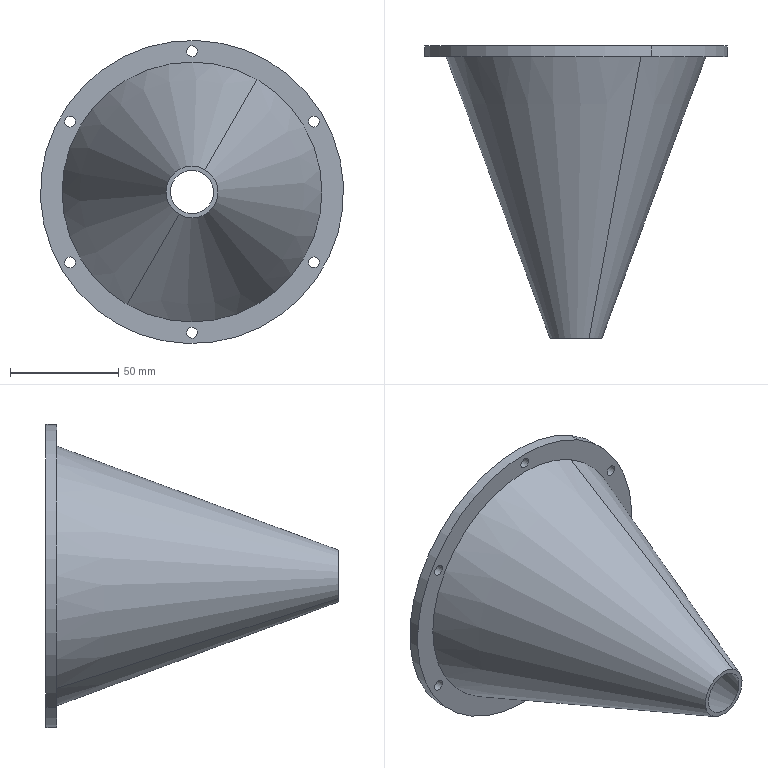Component | SolidWorks | WorkingHeadLowerCover-1 | 1 solid | 21 faces | box 140 x 135 x 140 mm | volume 112383 mm3 | cylinder 14 | cone 4 | plane 3 | commonest cylinder face diameters 5 x12 140 x2
build123d program:
from build123d import *

# Parameters (mm, degrees)
CUT_EXTRUDE1_REACH = 169.407
SKETCH2_R          = 2.5


with BuildPart() as part:
    # Sketch1 → Revolve1 (revolve)
    with BuildSketch(Plane.XY, mode=Mode.PRIVATE) as revolve1_sk:
        Polygon((-109.742, 0), (25.258, 0), (25.258, 12), (-104.742, 60), (-104.742, 70), (-109.742, 70), align=None)
    revolve(revolve1_sk.sketch.rotate(Axis((-109.742, 0, 0), (1, 0, 0)), 90), axis=Axis((-109.742, 0, 0), (1, 0, 0)))

    # Sketch2 → Cut-Extrude1 (cut, up to next)
    with BuildSketch(Plane.ZY.offset(109.742), mode=Mode.PRIVATE) as cut_extrude1_sk1:
        with Locations((0, 65)):
            Circle(SKETCH2_R)
    cut_extrude1_tool1 = extrude(cut_extrude1_sk1.sketch, amount=-CUT_EXTRUDE1_REACH, mode=Mode.PRIVATE) & part.part
    # Sketch2 → Cut-Extrude1 (cut, up to next)
    with BuildSketch(Plane.ZY.offset(109.742), mode=Mode.PRIVATE) as cut_extrude1_sk2:
        with Locations((56.292, 32.5)):
            Circle(SKETCH2_R)
    cut_extrude1_tool2 = extrude(cut_extrude1_sk2.sketch, amount=-CUT_EXTRUDE1_REACH, mode=Mode.PRIVATE) & part.part
    # Sketch2 → Cut-Extrude1 (cut, up to next)
    with BuildSketch(Plane.ZY.offset(109.742), mode=Mode.PRIVATE) as cut_extrude1_sk3:
        with Locations((56.292, -32.5)):
            Circle(SKETCH2_R)
    cut_extrude1_tool3 = extrude(cut_extrude1_sk3.sketch, amount=-CUT_EXTRUDE1_REACH, mode=Mode.PRIVATE) & part.part
    # Sketch2 → Cut-Extrude1 (cut, up to next)
    with BuildSketch(Plane.ZY.offset(109.742), mode=Mode.PRIVATE) as cut_extrude1_sk4:
        with Locations((0, -65)):
            Circle(SKETCH2_R)
    cut_extrude1_tool4 = extrude(cut_extrude1_sk4.sketch, amount=-CUT_EXTRUDE1_REACH, mode=Mode.PRIVATE) & part.part
    # Sketch2 → Cut-Extrude1 (cut, up to next)
    with BuildSketch(Plane.ZY.offset(109.742), mode=Mode.PRIVATE) as cut_extrude1_sk5:
        with Locations((-56.292, -32.5)):
            Circle(SKETCH2_R)
    cut_extrude1_tool5 = extrude(cut_extrude1_sk5.sketch, amount=-CUT_EXTRUDE1_REACH, mode=Mode.PRIVATE) & part.part
    # Sketch2 → Cut-Extrude1 (cut, up to next)
    with BuildSketch(Plane.ZY.offset(109.742), mode=Mode.PRIVATE) as cut_extrude1_sk6:
        with Locations((-56.292, 32.5)):
            Circle(SKETCH2_R)
    cut_extrude1_tool6 = extrude(cut_extrude1_sk6.sketch, amount=-CUT_EXTRUDE1_REACH, mode=Mode.PRIVATE) & part.part
    add(cut_extrude1_tool1.solids().sort_by_distance((-109.742, 65, 0))[0], mode=Mode.SUBTRACT)
    add(cut_extrude1_tool2.solids().sort_by_distance((-109.742, 32.5, 56.292))[0], mode=Mode.SUBTRACT)
    add(cut_extrude1_tool3.solids().sort_by_distance((-109.742, -32.5, 56.292))[0], mode=Mode.SUBTRACT)
    add(cut_extrude1_tool4.solids().sort_by_distance((-109.742, -65, 0))[0], mode=Mode.SUBTRACT)
    add(cut_extrude1_tool5.solids().sort_by_distance((-109.742, -32.5, -56.292))[0], mode=Mode.SUBTRACT)
    add(cut_extrude1_tool6.solids().sort_by_distance((-109.742, 32.5, -56.292))[0], mode=Mode.SUBTRACT)

    # Sketch3 → Cut-Revolve1 (revolve, cut)
    with BuildSketch(Plane(origin=(0, 0, 0), x_dir=(1, 0, 0), z_dir=(0, 1, 0)), mode=Mode.PRIVATE) as cut_revolve1_sk:
        Polygon((-109.742, 0), (25.258, 0), (25.258, 10), (-109.742, 58), align=None)
    revolve(cut_revolve1_sk.sketch.rotate(Axis((-109.742, 0, 0), (1, 0, 0)), 180), axis=Axis((-109.742, 0, 0), (1, 0, 0)), mode=Mode.SUBTRACT)


solid = part.part

# Placed as in the assembly
solid = solid.moved(Location((-5.981, -119.235, 160), (90, -90, 0)))
STEP:
#1=COLOUR_RGB('',0.7922,0.8196,0.9333);
#2=FILL_AREA_STYLE_COLOUR('',#1);
#3=FILL_AREA_STYLE('',(#2));
#4=SURFACE_STYLE_FILL_AREA(#3);
#5=SURFACE_SIDE_STYLE('',(#4));
#6=SURFACE_STYLE_USAGE(.BOTH.,#5);
#7=PRESENTATION_STYLE_ASSIGNMENT((#6));
#8=CARTESIAN_POINT('',(-0.4323,-5.689,5.958));
#9=VERTEX_POINT('',#8);
#10=CARTESIAN_POINT('',(-0.03862,-5.689,6.64));
#11=VERTEX_POINT('',#10);
#12=CARTESIAN_POINT('',(-0.2355,-5.689,6.299));
#13=DIRECTION('',(0.,1.,0.));
#14=DIRECTION('',(0.5,0.,0.866));
#15=AXIS2_PLACEMENT_3D('',#12,#13,#14);
#16=CIRCLE('',#15,0.3937);
#17=EDGE_CURVE('',#9,#11,#16,.T.);
#18=ORIENTED_EDGE('',*,*,#17,.F.);
#19=CARTESIAN_POINT('',(-1.377,-0.3738,4.322));
#20=VERTEX_POINT('',#19);
#21=CARTESIAN_POINT('',(-0.4323,-5.689,5.958));
#22=DIRECTION('',(-0.1675,0.9422,-0.2901));
#23=VECTOR('',#22,39.37);
#24=LINE('',#21,#23);
#25=EDGE_CURVE('',#9,#20,#24,.T.);
#26=ORIENTED_EDGE('',*,*,#25,.T.);
#27=CARTESIAN_POINT('',(0.9063,-0.3738,8.277));
#28=VERTEX_POINT('',#27);
#29=CARTESIAN_POINT('',(-0.2355,-0.3738,6.299));
#30=DIRECTION('',(0.,1.,0.));
#31=DIRECTION('',(0.5,0.,0.866));
#32=AXIS2_PLACEMENT_3D('',#29,#30,#31);
#33=CIRCLE('',#32,2.283);
#34=EDGE_CURVE('',#20,#28,#33,.T.);
#35=ORIENTED_EDGE('',*,*,#34,.T.);
#36=CARTESIAN_POINT('',(-0.03862,-5.689,6.64));
#37=DIRECTION('',(0.1675,0.9422,0.2901));
#38=VECTOR('',#37,39.37);
#39=LINE('',#36,#38);
#40=EDGE_CURVE('',#11,#28,#39,.T.);
#41=ORIENTED_EDGE('',*,*,#40,.F.);
#42=EDGE_LOOP('',(#18,#26,#35,#41));
#43=FACE_OUTER_BOUND('',#42,.T.);
#44=CARTESIAN_POINT('',(-0.2355,-5.689,6.299));
#45=DIRECTION('',(0.,1.,0.));
#46=DIRECTION('',(0.5,0.,0.866));
#47=AXIS2_PLACEMENT_3D('',#44,#45,#46);
#48=CONICAL_SURFACE('',#47,0.3937,0.3416);
#49=ADVANCED_FACE('',(#43),#48,.F.);
#50=CARTESIAN_POINT('',(2.03,-0.5706,5.105));
#51=VERTEX_POINT('',#50);
#52=CARTESIAN_POINT('',(1.932,-0.5706,4.934));
#53=VERTEX_POINT('',#52);
#54=CARTESIAN_POINT('',(1.981,-0.5706,5.02));
#55=DIRECTION('',(0.,-1.,0.));
#56=DIRECTION('',(0.5,0.,0.866));
#57=AXIS2_PLACEMENT_3D('',#54,#55,#56);
#58=CIRCLE('',#57,0.09843);
#59=EDGE_CURVE('',#51,#53,#58,.T.);
#60=ORIENTED_EDGE('',*,*,#59,.T.);
#61=CARTESIAN_POINT('',(1.932,-0.3738,4.934));
#62=VERTEX_POINT('',#61);
#63=CARTESIAN_POINT('',(1.932,-5.689,4.934));
#64=DIRECTION('',(0.,1.,0.));
#65=VECTOR('',#64,39.37);
#66=LINE('',#63,#65);
#67=EDGE_CURVE('',#53,#62,#66,.T.);
#68=ORIENTED_EDGE('',*,*,#67,.T.);
#69=CARTESIAN_POINT('',(2.03,-0.3738,5.105));
#70=VERTEX_POINT('',#69);
#71=CARTESIAN_POINT('',(1.981,-0.3738,5.02));
#72=DIRECTION('',(0.,1.,0.));
#73=DIRECTION('',(0.5,0.,0.866));
#74=AXIS2_PLACEMENT_3D('',#71,#72,#73);
#75=CIRCLE('',#74,0.09843);
#76=EDGE_CURVE('',#62,#70,#75,.T.);
#77=ORIENTED_EDGE('',*,*,#76,.T.);
#78=CARTESIAN_POINT('',(2.03,-5.689,5.105));
#79=DIRECTION('',(0.,1.,0.));
#80=VECTOR('',#79,39.37);
#81=LINE('',#78,#80);
#82=EDGE_CURVE('',#51,#70,#81,.T.);
#83=ORIENTED_EDGE('',*,*,#82,.F.);
#84=EDGE_LOOP('',(#60,#68,#77,#83));
#85=FACE_OUTER_BOUND('',#84,.T.);
#86=CARTESIAN_POINT('',(1.981,-5.689,5.02));
#87=DIRECTION('',(0.,1.,0.));
#88=DIRECTION('',(0.5,0.,0.866));
#89=AXIS2_PLACEMENT_3D('',#86,#87,#88);
#90=CYLINDRICAL_SURFACE('',#89,0.09843);
#91=ADVANCED_FACE('',(#85),#90,.F.);
#92=CARTESIAN_POINT('',(-0.1863,-0.5706,3.825));
#93=VERTEX_POINT('',#92);
#94=CARTESIAN_POINT('',(-0.2847,-0.5706,3.655));
#95=VERTEX_POINT('',#94);
#96=CARTESIAN_POINT('',(-0.2355,-0.5706,3.74));
#97=DIRECTION('',(0.,-1.,0.));
#98=DIRECTION('',(0.5,0.,0.866));
#99=AXIS2_PLACEMENT_3D('',#96,#97,#98);
#100=CIRCLE('',#99,0.09843);
#101=EDGE_CURVE('',#93,#95,#100,.T.);
#102=ORIENTED_EDGE('',*,*,#101,.T.);
#103=CARTESIAN_POINT('',(-0.2847,-0.3738,3.655));
#104=VERTEX_POINT('',#103);
#105=CARTESIAN_POINT('',(-0.2847,-5.689,3.655));
#106=DIRECTION('',(0.,1.,0.));
#107=VECTOR('',#106,39.37);
#108=LINE('',#105,#107);
#109=EDGE_CURVE('',#95,#104,#108,.T.);
#110=ORIENTED_EDGE('',*,*,#109,.T.);
#111=CARTESIAN_POINT('',(-0.1863,-0.3738,3.825));
#112=VERTEX_POINT('',#111);
#113=CARTESIAN_POINT('',(-0.2355,-0.3738,3.74));
#114=DIRECTION('',(0.,1.,0.));
#115=DIRECTION('',(0.5,0.,0.866));
#116=AXIS2_PLACEMENT_3D('',#113,#114,#115);
#117=CIRCLE('',#116,0.09843);
#118=EDGE_CURVE('',#104,#112,#117,.T.);
#119=ORIENTED_EDGE('',*,*,#118,.T.);
#120=CARTESIAN_POINT('',(-0.1863,-5.689,3.825));
#121=DIRECTION('',(0.,1.,0.));
#122=VECTOR('',#121,39.37);
#123=LINE('',#120,#122);
#124=EDGE_CURVE('',#93,#112,#123,.T.);
#125=ORIENTED_EDGE('',*,*,#124,.F.);
#126=EDGE_LOOP('',(#102,#110,#119,#125));
#127=FACE_OUTER_BOUND('',#126,.T.);
#128=CARTESIAN_POINT('',(-0.2355,-5.689,3.74));
#129=DIRECTION('',(0.,1.,0.));
#130=DIRECTION('',(0.5,0.,0.866));
#131=AXIS2_PLACEMENT_3D('',#128,#129,#130);
#132=CYLINDRICAL_SURFACE('',#131,0.09843);
#133=ADVANCED_FACE('',(#127),#132,.F.);
#134=CARTESIAN_POINT('',(-2.402,-0.5706,5.105));
#135=VERTEX_POINT('',#134);
#136=CARTESIAN_POINT('',(-2.501,-0.5706,4.934));
#137=VERTEX_POINT('',#136);
#138=CARTESIAN_POINT('',(-2.452,-0.5706,5.02));
#139=DIRECTION('',(0.,-1.,0.));
#140=DIRECTION('',(0.5,0.,0.866));
#141=AXIS2_PLACEMENT_3D('',#138,#139,#140);
#142=CIRCLE('',#141,0.09843);
#143=EDGE_CURVE('',#135,#137,#142,.T.);
#144=ORIENTED_EDGE('',*,*,#143,.T.);
#145=CARTESIAN_POINT('',(-2.501,-0.3738,4.934));
#146=VERTEX_POINT('',#145);
#147=CARTESIAN_POINT('',(-2.501,-5.689,4.934));
#148=DIRECTION('',(0.,1.,0.));
#149=VECTOR('',#148,39.37);
#150=LINE('',#147,#149);
#151=EDGE_CURVE('',#137,#146,#150,.T.);
#152=ORIENTED_EDGE('',*,*,#151,.T.);
#153=CARTESIAN_POINT('',(-2.402,-0.3738,5.105));
#154=VERTEX_POINT('',#153);
#155=CARTESIAN_POINT('',(-2.452,-0.3738,5.02));
#156=DIRECTION('',(0.,1.,0.));
#157=DIRECTION('',(0.5,0.,0.866));
#158=AXIS2_PLACEMENT_3D('',#155,#156,#157);
#159=CIRCLE('',#158,0.09843);
#160=EDGE_CURVE('',#146,#154,#159,.T.);
#161=ORIENTED_EDGE('',*,*,#160,.T.);
#162=CARTESIAN_POINT('',(-2.402,-5.689,5.105));
#163=DIRECTION('',(0.,1.,0.));
#164=VECTOR('',#163,39.37);
#165=LINE('',#162,#164);
#166=EDGE_CURVE('',#135,#154,#165,.T.);
#167=ORIENTED_EDGE('',*,*,#166,.F.);
#168=EDGE_LOOP('',(#144,#152,#161,#167));
#169=FACE_OUTER_BOUND('',#168,.T.);
#170=CARTESIAN_POINT('',(-2.452,-5.689,5.02));
#171=DIRECTION('',(0.,1.,0.));
#172=DIRECTION('',(0.5,0.,0.866));
#173=AXIS2_PLACEMENT_3D('',#170,#171,#172);
#174=CYLINDRICAL_SURFACE('',#173,0.09843);
#175=ADVANCED_FACE('',(#169),#174,.F.);
#176=CARTESIAN_POINT('',(-2.402,-0.5706,7.664));
#177=VERTEX_POINT('',#176);
#178=CARTESIAN_POINT('',(-2.501,-0.5706,7.494));
#179=VERTEX_POINT('',#178);
#180=CARTESIAN_POINT('',(-2.452,-0.5706,7.579));
#181=DIRECTION('',(0.,-1.,0.));
#182=DIRECTION('',(0.5,0.,0.866));
#183=AXIS2_PLACEMENT_3D('',#180,#181,#182);
#184=CIRCLE('',#183,0.09843);
#185=EDGE_CURVE('',#177,#179,#184,.T.);
#186=ORIENTED_EDGE('',*,*,#185,.T.);
#187=CARTESIAN_POINT('',(-2.501,-0.3738,7.494));
#188=VERTEX_POINT('',#187);
#189=CARTESIAN_POINT('',(-2.501,-5.689,7.494));
#190=DIRECTION('',(0.,1.,0.));
#191=VECTOR('',#190,39.37);
#192=LINE('',#189,#191);
#193=EDGE_CURVE('',#179,#188,#192,.T.);
#194=ORIENTED_EDGE('',*,*,#193,.T.);
#195=CARTESIAN_POINT('',(-2.402,-0.3738,7.664));
#196=VERTEX_POINT('',#195);
#197=CARTESIAN_POINT('',(-2.452,-0.3738,7.579));
#198=DIRECTION('',(0.,1.,0.));
#199=DIRECTION('',(0.5,0.,0.866));
#200=AXIS2_PLACEMENT_3D('',#197,#198,#199);
#201=CIRCLE('',#200,0.09843);
#202=EDGE_CURVE('',#188,#196,#201,.T.);
#203=ORIENTED_EDGE('',*,*,#202,.T.);
#204=CARTESIAN_POINT('',(-2.402,-5.689,7.664));
#205=DIRECTION('',(0.,1.,0.));
#206=VECTOR('',#205,39.37);
#207=LINE('',#204,#206);
#208=EDGE_CURVE('',#177,#196,#207,.T.);
#209=ORIENTED_EDGE('',*,*,#208,.F.);
#210=EDGE_LOOP('',(#186,#194,#203,#209));
#211=FACE_OUTER_BOUND('',#210,.T.);
#212=CARTESIAN_POINT('',(-2.452,-5.689,7.579));
#213=DIRECTION('',(0.,1.,0.));
#214=DIRECTION('',(0.5,0.,0.866));
#215=AXIS2_PLACEMENT_3D('',#212,#213,#214);
#216=CYLINDRICAL_SURFACE('',#215,0.09843);
#217=ADVANCED_FACE('',(#211),#216,.F.);
#218=CARTESIAN_POINT('',(-0.1863,-0.5706,8.944));
#219=VERTEX_POINT('',#218);
#220=CARTESIAN_POINT('',(-0.2847,-0.5706,8.773));
#221=VERTEX_POINT('',#220);
#222=CARTESIAN_POINT('',(-0.2355,-0.5706,8.858));
#223=DIRECTION('',(0.,-1.,0.));
#224=DIRECTION('',(0.5,0.,0.866));
#225=AXIS2_PLACEMENT_3D('',#222,#223,#224);
#226=CIRCLE('',#225,0.09843);
#227=EDGE_CURVE('',#219,#221,#226,.T.);
#228=ORIENTED_EDGE('',*,*,#227,.T.);
#229=CARTESIAN_POINT('',(-0.2847,-0.3738,8.773));
#230=VERTEX_POINT('',#229);
#231=CARTESIAN_POINT('',(-0.2847,-5.689,8.773));
#232=DIRECTION('',(0.,1.,0.));
#233=VECTOR('',#232,39.37);
#234=LINE('',#231,#233);
#235=EDGE_CURVE('',#221,#230,#234,.T.);
#236=ORIENTED_EDGE('',*,*,#235,.T.);
#237=CARTESIAN_POINT('',(-0.1863,-0.3738,8.944));
#238=VERTEX_POINT('',#237);
#239=CARTESIAN_POINT('',(-0.2355,-0.3738,8.858));
#240=DIRECTION('',(0.,1.,0.));
#241=DIRECTION('',(0.5,0.,0.866));
#242=AXIS2_PLACEMENT_3D('',#239,#240,#241);
#243=CIRCLE('',#242,0.09843);
#244=EDGE_CURVE('',#230,#238,#243,.T.);
#245=ORIENTED_EDGE('',*,*,#244,.T.);
#246=CARTESIAN_POINT('',(-0.1863,-5.689,8.944));
#247=DIRECTION('',(0.,1.,0.));
#248=VECTOR('',#247,39.37);
#249=LINE('',#246,#248);
#250=EDGE_CURVE('',#219,#238,#249,.T.);
#251=ORIENTED_EDGE('',*,*,#250,.F.);
#252=EDGE_LOOP('',(#228,#236,#245,#251));
#253=FACE_OUTER_BOUND('',#252,.T.);
#254=CARTESIAN_POINT('',(-0.2355,-5.689,8.858));
#255=DIRECTION('',(0.,1.,0.));
#256=DIRECTION('',(0.5,0.,0.866));
#257=AXIS2_PLACEMENT_3D('',#254,#255,#256);
#258=CYLINDRICAL_SURFACE('',#257,0.09843);
#259=ADVANCED_FACE('',(#253),#258,.F.);
#260=CARTESIAN_POINT('',(2.03,-0.5706,7.664));
#261=VERTEX_POINT('',#260);
#262=CARTESIAN_POINT('',(1.932,-0.5706,7.494));
#263=VERTEX_POINT('',#262);
#264=CARTESIAN_POINT('',(1.981,-0.5706,7.579));
#265=DIRECTION('',(0.,-1.,0.));
#266=DIRECTION('',(0.5,0.,0.866));
#267=AXIS2_PLACEMENT_3D('',#264,#265,#266);
#268=CIRCLE('',#267,0.09843);
#269=EDGE_CURVE('',#261,#263,#268,.T.);
#270=ORIENTED_EDGE('',*,*,#269,.T.);
#271=CARTESIAN_POINT('',(1.932,-0.3738,7.494));
#272=VERTEX_POINT('',#271);
#273=CARTESIAN_POINT('',(1.932,-5.689,7.494));
#274=DIRECTION('',(0.,1.,0.));
#275=VECTOR('',#274,39.37);
#276=LINE('',#273,#275);
#277=EDGE_CURVE('',#263,#272,#276,.T.);
#278=ORIENTED_EDGE('',*,*,#277,.T.);
#279=CARTESIAN_POINT('',(2.03,-0.3738,7.664));
#280=VERTEX_POINT('',#279);
#281=CARTESIAN_POINT('',(1.981,-0.3738,7.579));
#282=DIRECTION('',(0.,1.,0.));
#283=DIRECTION('',(0.5,0.,0.866));
#284=AXIS2_PLACEMENT_3D('',#281,#282,#283);
#285=CIRCLE('',#284,0.09843);
#286=EDGE_CURVE('',#272,#280,#285,.T.);
#287=ORIENTED_EDGE('',*,*,#286,.T.);
#288=CARTESIAN_POINT('',(2.03,-5.689,7.664));
#289=DIRECTION('',(0.,1.,0.));
#290=VECTOR('',#289,39.37);
#291=LINE('',#288,#290);
#292=EDGE_CURVE('',#261,#280,#291,.T.);
#293=ORIENTED_EDGE('',*,*,#292,.F.);
#294=EDGE_LOOP('',(#270,#278,#287,#293));
#295=FACE_OUTER_BOUND('',#294,.T.);
#296=CARTESIAN_POINT('',(1.981,-5.689,7.579));
#297=DIRECTION('',(0.,1.,0.));
#298=DIRECTION('',(0.5,0.,0.866));
#299=AXIS2_PLACEMENT_3D('',#296,#297,#298);
#300=CYLINDRICAL_SURFACE('',#299,0.09843);
#301=ADVANCED_FACE('',(#295),#300,.F.);
#302=CARTESIAN_POINT('',(1.142,-0.5706,8.686));
#303=VERTEX_POINT('',#302);
#304=CARTESIAN_POINT('',(-1.613,-0.5706,3.913));
#305=VERTEX_POINT('',#304);
#306=CARTESIAN_POINT('',(-0.2355,-0.5706,6.299));
#307=DIRECTION('',(0.,1.,0.));
#308=DIRECTION('',(0.5,0.,0.866));
#309=AXIS2_PLACEMENT_3D('',#306,#307,#308);
#310=CIRCLE('',#309,2.756);
#311=EDGE_CURVE('',#303,#305,#310,.T.);
#312=ORIENTED_EDGE('',*,*,#311,.T.);
#313=CARTESIAN_POINT('',(-1.613,-0.3738,3.913));
#314=VERTEX_POINT('',#313);
#315=CARTESIAN_POINT('',(-1.613,-0.3738,3.913));
#316=DIRECTION('',(0.,1.,0.));
#317=VECTOR('',#316,39.37);
#318=LINE('',#315,#317);
#319=EDGE_CURVE('',#305,#314,#318,.T.);
#320=ORIENTED_EDGE('',*,*,#319,.T.);
#321=CARTESIAN_POINT('',(1.142,-0.3738,8.686));
#322=VERTEX_POINT('',#321);
#323=CARTESIAN_POINT('',(-0.2355,-0.3738,6.299));
#324=DIRECTION('',(0.,1.,0.));
#325=DIRECTION('',(0.5,0.,0.866));
#326=AXIS2_PLACEMENT_3D('',#323,#324,#325);
#327=CIRCLE('',#326,2.756);
#328=EDGE_CURVE('',#322,#314,#327,.T.);
#329=ORIENTED_EDGE('',*,*,#328,.F.);
#330=CARTESIAN_POINT('',(1.142,-0.3738,8.686));
#331=DIRECTION('',(0.,1.,0.));
#332=VECTOR('',#331,39.37);
#333=LINE('',#330,#332);
#334=EDGE_CURVE('',#303,#322,#333,.T.);
#335=ORIENTED_EDGE('',*,*,#334,.F.);
#336=EDGE_LOOP('',(#312,#320,#329,#335));
#337=FACE_OUTER_BOUND('',#336,.T.);
#338=CARTESIAN_POINT('',(-0.2355,-0.3738,6.299));
#339=DIRECTION('',(0.,1.,0.));
#340=DIRECTION('',(0.5,0.,0.866));
#341=AXIS2_PLACEMENT_3D('',#338,#339,#340);
#342=CYLINDRICAL_SURFACE('',#341,2.756);
#343=ADVANCED_FACE('',(#337),#342,.T.);
#344=CARTESIAN_POINT('',(0.0007521,-5.689,6.708));
#345=VERTEX_POINT('',#344);
#346=CARTESIAN_POINT('',(-0.4717,-5.689,5.89));
#347=VERTEX_POINT('',#346);
#348=CARTESIAN_POINT('',(-0.2355,-5.689,6.299));
#349=DIRECTION('',(0.,1.,0.));
#350=DIRECTION('',(0.5,0.,0.866));
#351=AXIS2_PLACEMENT_3D('',#348,#349,#350);
#352=CIRCLE('',#351,0.4724);
#353=EDGE_CURVE('',#345,#347,#352,.T.);
#354=ORIENTED_EDGE('',*,*,#353,.T.);
#355=CARTESIAN_POINT('',(-1.417,-0.5706,4.253));
#356=VERTEX_POINT('',#355);
#357=CARTESIAN_POINT('',(-0.4717,-5.689,5.89));
#358=DIRECTION('',(-0.1732,0.9381,-0.3));
#359=VECTOR('',#358,39.37);
#360=LINE('',#357,#359);
#361=EDGE_CURVE('',#347,#356,#360,.T.);
#362=ORIENTED_EDGE('',*,*,#361,.T.);
#363=CARTESIAN_POINT('',(0.9456,-0.5706,8.345));
#364=VERTEX_POINT('',#363);
#365=CARTESIAN_POINT('',(-0.2355,-0.5706,6.299));
#366=DIRECTION('',(0.,1.,0.));
#367=DIRECTION('',(0.5,0.,0.866));
#368=AXIS2_PLACEMENT_3D('',#365,#366,#367);
#369=CIRCLE('',#368,2.362);
#370=EDGE_CURVE('',#364,#356,#369,.T.);
#371=ORIENTED_EDGE('',*,*,#370,.F.);
#372=CARTESIAN_POINT('',(0.0007521,-5.689,6.708));
#373=DIRECTION('',(0.1732,0.9381,0.3));
#374=VECTOR('',#373,39.37);
#375=LINE('',#372,#374);
#376=EDGE_CURVE('',#345,#364,#375,.T.);
#377=ORIENTED_EDGE('',*,*,#376,.F.);
#378=EDGE_LOOP('',(#354,#362,#371,#377));
#379=FACE_OUTER_BOUND('',#378,.T.);
#380=CARTESIAN_POINT('',(-0.2355,-5.689,6.299));
#381=DIRECTION('',(0.,1.,0.));
#382=DIRECTION('',(0.5,0.,0.866));
#383=AXIS2_PLACEMENT_3D('',#380,#381,#382);
#384=CONICAL_SURFACE('',#383,0.4724,0.3537);
#385=ADVANCED_FACE('',(#379),#384,.T.);
#386=CARTESIAN_POINT('',(-0.2355,-0.3738,6.299));
#387=DIRECTION('',(0.,1.,0.));
#388=DIRECTION('',(0.5,0.,0.866));
#389=AXIS2_PLACEMENT_3D('',#386,#387,#388);
#390=CIRCLE('',#389,2.283);
#391=EDGE_CURVE('',#28,#20,#390,.T.);
#392=ORIENTED_EDGE('',*,*,#391,.F.);
#393=ORIENTED_EDGE('',*,*,#34,.F.);
#394=EDGE_LOOP('',(#392,#393));
#395=FACE_BOUND('',#394,.T.);
#396=CARTESIAN_POINT('',(1.981,-0.3738,5.02));
#397=DIRECTION('',(0.,1.,0.));
#398=DIRECTION('',(0.5,0.,0.866));
#399=AXIS2_PLACEMENT_3D('',#396,#397,#398);
#400=CIRCLE('',#399,0.09843);
#401=EDGE_CURVE('',#70,#62,#400,.T.);
#402=ORIENTED_EDGE('',*,*,#401,.F.);
#403=ORIENTED_EDGE('',*,*,#76,.F.);
#404=EDGE_LOOP('',(#402,#403));
#405=FACE_BOUND('',#404,.T.);
#406=CARTESIAN_POINT('',(-0.2355,-0.3738,3.74));
#407=DIRECTION('',(0.,1.,0.));
#408=DIRECTION('',(0.5,0.,0.866));
#409=AXIS2_PLACEMENT_3D('',#406,#407,#408);
#410=CIRCLE('',#409,0.09843);
#411=EDGE_CURVE('',#112,#104,#410,.T.);
#412=ORIENTED_EDGE('',*,*,#411,.F.);
#413=ORIENTED_EDGE('',*,*,#118,.F.);
#414=EDGE_LOOP('',(#412,#413));
#415=FACE_BOUND('',#414,.T.);
#416=CARTESIAN_POINT('',(-2.452,-0.3738,5.02));
#417=DIRECTION('',(0.,1.,0.));
#418=DIRECTION('',(0.5,0.,0.866));
#419=AXIS2_PLACEMENT_3D('',#416,#417,#418);
#420=CIRCLE('',#419,0.09843);
#421=EDGE_CURVE('',#154,#146,#420,.T.);
#422=ORIENTED_EDGE('',*,*,#421,.F.);
#423=ORIENTED_EDGE('',*,*,#160,.F.);
#424=EDGE_LOOP('',(#422,#423));
#425=FACE_BOUND('',#424,.T.);
#426=CARTESIAN_POINT('',(-2.452,-0.3738,7.579));
#427=DIRECTION('',(0.,1.,0.));
#428=DIRECTION('',(0.5,0.,0.866));
#429=AXIS2_PLACEMENT_3D('',#426,#427,#428);
#430=CIRCLE('',#429,0.09843);
#431=EDGE_CURVE('',#196,#188,#430,.T.);
#432=ORIENTED_EDGE('',*,*,#431,.F.);
#433=ORIENTED_EDGE('',*,*,#202,.F.);
#434=EDGE_LOOP('',(#432,#433));
#435=FACE_BOUND('',#434,.T.);
#436=CARTESIAN_POINT('',(-0.2355,-0.3738,8.858));
#437=DIRECTION('',(0.,1.,0.));
#438=DIRECTION('',(0.5,0.,0.866));
#439=AXIS2_PLACEMENT_3D('',#436,#437,#438);
#440=CIRCLE('',#439,0.09843);
#441=EDGE_CURVE('',#238,#230,#440,.T.);
#442=ORIENTED_EDGE('',*,*,#441,.F.);
#443=ORIENTED_EDGE('',*,*,#244,.F.);
#444=EDGE_LOOP('',(#442,#443));
#445=FACE_BOUND('',#444,.T.);
#446=CARTESIAN_POINT('',(1.981,-0.3738,7.579));
#447=DIRECTION('',(0.,1.,0.));
#448=DIRECTION('',(0.5,0.,0.866));
#449=AXIS2_PLACEMENT_3D('',#446,#447,#448);
#450=CIRCLE('',#449,0.09843);
#451=EDGE_CURVE('',#280,#272,#450,.T.);
#452=ORIENTED_EDGE('',*,*,#451,.F.);
#453=ORIENTED_EDGE('',*,*,#286,.F.);
#454=EDGE_LOOP('',(#452,#453));
#455=FACE_BOUND('',#454,.T.);
#456=ORIENTED_EDGE('',*,*,#328,.T.);
#457=CARTESIAN_POINT('',(-0.2355,-0.3738,6.299));
#458=DIRECTION('',(0.,1.,0.));
#459=DIRECTION('',(0.5,0.,0.866));
#460=AXIS2_PLACEMENT_3D('',#457,#458,#459);
#461=CIRCLE('',#460,2.756);
#462=EDGE_CURVE('',#314,#322,#461,.T.);
#463=ORIENTED_EDGE('',*,*,#462,.T.);
#464=EDGE_LOOP('',(#456,#463));
#465=FACE_OUTER_BOUND('',#464,.T.);
#466=CARTESIAN_POINT('',(2.151,-0.3738,4.921));
#467=DIRECTION('',(0.,-1.,0.));
#468=DIRECTION('',(-0.5,0.,-0.866));
#469=AXIS2_PLACEMENT_3D('',#466,#467,#468);
#470=PLANE('',#469);
#471=ADVANCED_FACE('',(#395,#405,#415,#425,#435,#445,#455,#465),#470,.F.);
#472=CARTESIAN_POINT('',(-0.2355,-5.689,6.299));
#473=DIRECTION('',(0.,1.,0.));
#474=DIRECTION('',(0.5,0.,0.866));
#475=AXIS2_PLACEMENT_3D('',#472,#473,#474);
#476=CIRCLE('',#475,0.3937);
#477=EDGE_CURVE('',#11,#9,#476,.T.);
#478=ORIENTED_EDGE('',*,*,#477,.T.);
#479=ORIENTED_EDGE('',*,*,#17,.T.);
#480=EDGE_LOOP('',(#478,#479));
#481=FACE_BOUND('',#480,.T.);
#482=ORIENTED_EDGE('',*,*,#353,.F.);
#483=CARTESIAN_POINT('',(-0.2355,-5.689,6.299));
#484=DIRECTION('',(0.,1.,0.));
#485=DIRECTION('',(0.5,0.,0.866));
#486=AXIS2_PLACEMENT_3D('',#483,#484,#485);
#487=CIRCLE('',#486,0.4724);
#488=EDGE_CURVE('',#347,#345,#487,.T.);
#489=ORIENTED_EDGE('',*,*,#488,.F.);
#490=EDGE_LOOP('',(#482,#489));
#491=FACE_OUTER_BOUND('',#490,.T.);
#492=CARTESIAN_POINT('',(-0.2355,-5.689,6.299));
#493=DIRECTION('',(0.,1.,0.));
#494=DIRECTION('',(0.5,0.,0.866));
#495=AXIS2_PLACEMENT_3D('',#492,#493,#494);
#496=PLANE('',#495);
#497=ADVANCED_FACE('',(#481,#491),#496,.F.);
#498=ORIENTED_EDGE('',*,*,#361,.F.);
#499=ORIENTED_EDGE('',*,*,#488,.T.);
#500=ORIENTED_EDGE('',*,*,#376,.T.);
#501=CARTESIAN_POINT('',(-0.2355,-0.5706,6.299));
#502=DIRECTION('',(0.,1.,0.));
#503=DIRECTION('',(0.5,0.,0.866));
#504=AXIS2_PLACEMENT_3D('',#501,#502,#503);
#505=CIRCLE('',#504,2.362);
#506=EDGE_CURVE('',#356,#364,#505,.T.);
#507=ORIENTED_EDGE('',*,*,#506,.F.);
#508=EDGE_LOOP('',(#498,#499,#500,#507));
#509=FACE_OUTER_BOUND('',#508,.T.);
#510=CARTESIAN_POINT('',(-0.2355,-5.689,6.299));
#511=DIRECTION('',(0.,1.,0.));
#512=DIRECTION('',(0.5,0.,0.866));
#513=AXIS2_PLACEMENT_3D('',#510,#511,#512);
#514=CONICAL_SURFACE('',#513,0.4724,0.3537);
#515=ADVANCED_FACE('',(#509),#514,.T.);
#516=ORIENTED_EDGE('',*,*,#59,.F.);
#517=CARTESIAN_POINT('',(1.981,-0.5706,5.02));
#518=DIRECTION('',(0.,-1.,0.));
#519=DIRECTION('',(0.5,0.,0.866));
#520=AXIS2_PLACEMENT_3D('',#517,#518,#519);
#521=CIRCLE('',#520,0.09843);
#522=EDGE_CURVE('',#53,#51,#521,.T.);
#523=ORIENTED_EDGE('',*,*,#522,.F.);
#524=EDGE_LOOP('',(#516,#523));
#525=FACE_BOUND('',#524,.T.);
#526=ORIENTED_EDGE('',*,*,#101,.F.);
#527=CARTESIAN_POINT('',(-0.2355,-0.5706,3.74));
#528=DIRECTION('',(0.,-1.,0.));
#529=DIRECTION('',(0.5,0.,0.866));
#530=AXIS2_PLACEMENT_3D('',#527,#528,#529);
#531=CIRCLE('',#530,0.09843);
#532=EDGE_CURVE('',#95,#93,#531,.T.);
#533=ORIENTED_EDGE('',*,*,#532,.F.);
#534=EDGE_LOOP('',(#526,#533));
#535=FACE_BOUND('',#534,.T.);
#536=ORIENTED_EDGE('',*,*,#143,.F.);
#537=CARTESIAN_POINT('',(-2.452,-0.5706,5.02));
#538=DIRECTION('',(0.,-1.,0.));
#539=DIRECTION('',(0.5,0.,0.866));
#540=AXIS2_PLACEMENT_3D('',#537,#538,#539);
#541=CIRCLE('',#540,0.09843);
#542=EDGE_CURVE('',#137,#135,#541,.T.);
#543=ORIENTED_EDGE('',*,*,#542,.F.);
#544=EDGE_LOOP('',(#536,#543));
#545=FACE_BOUND('',#544,.T.);
#546=ORIENTED_EDGE('',*,*,#185,.F.);
#547=CARTESIAN_POINT('',(-2.452,-0.5706,7.579));
#548=DIRECTION('',(0.,-1.,0.));
#549=DIRECTION('',(0.5,0.,0.866));
#550=AXIS2_PLACEMENT_3D('',#547,#548,#549);
#551=CIRCLE('',#550,0.09843);
#552=EDGE_CURVE('',#179,#177,#551,.T.);
#553=ORIENTED_EDGE('',*,*,#552,.F.);
#554=EDGE_LOOP('',(#546,#553));
#555=FACE_BOUND('',#554,.T.);
#556=ORIENTED_EDGE('',*,*,#227,.F.);
#557=CARTESIAN_POINT('',(-0.2355,-0.5706,8.858));
#558=DIRECTION('',(0.,-1.,0.));
#559=DIRECTION('',(0.5,0.,0.866));
#560=AXIS2_PLACEMENT_3D('',#557,#558,#559);
#561=CIRCLE('',#560,0.09843);
#562=EDGE_CURVE('',#221,#219,#561,.T.);
#563=ORIENTED_EDGE('',*,*,#562,.F.);
#564=EDGE_LOOP('',(#556,#563));
#565=FACE_BOUND('',#564,.T.);
#566=ORIENTED_EDGE('',*,*,#269,.F.);
#567=CARTESIAN_POINT('',(1.981,-0.5706,7.579));
#568=DIRECTION('',(0.,-1.,0.));
#569=DIRECTION('',(0.5,0.,0.866));
#570=AXIS2_PLACEMENT_3D('',#567,#568,#569);
#571=CIRCLE('',#570,0.09843);
#572=EDGE_CURVE('',#263,#261,#571,.T.);
#573=ORIENTED_EDGE('',*,*,#572,.F.);
#574=EDGE_LOOP('',(#566,#573));
#575=FACE_BOUND('',#574,.T.);
#576=ORIENTED_EDGE('',*,*,#311,.F.);
#577=CARTESIAN_POINT('',(-0.2355,-0.5706,6.299));
#578=DIRECTION('',(0.,1.,0.));
#579=DIRECTION('',(0.5,0.,0.866));
#580=AXIS2_PLACEMENT_3D('',#577,#578,#579);
#581=CIRCLE('',#580,2.756);
#582=EDGE_CURVE('',#305,#303,#581,.T.);
#583=ORIENTED_EDGE('',*,*,#582,.F.);
#584=EDGE_LOOP('',(#576,#583));
#585=FACE_OUTER_BOUND('',#584,.T.);
#586=ORIENTED_EDGE('',*,*,#370,.T.);
#587=ORIENTED_EDGE('',*,*,#506,.T.);
#588=EDGE_LOOP('',(#586,#587));
#589=FACE_BOUND('',#588,.T.);
#590=CARTESIAN_POINT('',(1.81,-0.5706,5.118));
#591=DIRECTION('',(0.,1.,0.));
#592=DIRECTION('',(0.5,0.,0.866));
#593=AXIS2_PLACEMENT_3D('',#590,#591,#592);
#594=PLANE('',#593);
#595=ADVANCED_FACE('',(#525,#535,#545,#555,#565,#575,#585,#589),#594,.F.);
#596=ORIENTED_EDGE('',*,*,#319,.F.);
#597=ORIENTED_EDGE('',*,*,#582,.T.);
#598=ORIENTED_EDGE('',*,*,#334,.T.);
#599=ORIENTED_EDGE('',*,*,#462,.F.);
#600=EDGE_LOOP('',(#596,#597,#598,#599));
#601=FACE_OUTER_BOUND('',#600,.T.);
#602=CARTESIAN_POINT('',(-0.2355,-0.3738,6.299));
#603=DIRECTION('',(0.,1.,0.));
#604=DIRECTION('',(0.5,0.,0.866));
#605=AXIS2_PLACEMENT_3D('',#602,#603,#604);
#606=CYLINDRICAL_SURFACE('',#605,2.756);
#607=ADVANCED_FACE('',(#601),#606,.T.);
#608=ORIENTED_EDGE('',*,*,#277,.F.);
#609=ORIENTED_EDGE('',*,*,#572,.T.);
#610=ORIENTED_EDGE('',*,*,#292,.T.);
#611=ORIENTED_EDGE('',*,*,#451,.T.);
#612=EDGE_LOOP('',(#608,#609,#610,#611));
#613=FACE_OUTER_BOUND('',#612,.T.);
#614=CARTESIAN_POINT('',(1.981,-5.689,7.579));
#615=DIRECTION('',(0.,1.,0.));
#616=DIRECTION('',(0.5,0.,0.866));
#617=AXIS2_PLACEMENT_3D('',#614,#615,#616);
#618=CYLINDRICAL_SURFACE('',#617,0.09843);
#619=ADVANCED_FACE('',(#613),#618,.F.);
#620=ORIENTED_EDGE('',*,*,#235,.F.);
#621=ORIENTED_EDGE('',*,*,#562,.T.);
#622=ORIENTED_EDGE('',*,*,#250,.T.);
#623=ORIENTED_EDGE('',*,*,#441,.T.);
#624=EDGE_LOOP('',(#620,#621,#622,#623));
#625=FACE_OUTER_BOUND('',#624,.T.);
#626=CARTESIAN_POINT('',(-0.2355,-5.689,8.858));
#627=DIRECTION('',(0.,1.,0.));
#628=DIRECTION('',(0.5,0.,0.866));
#629=AXIS2_PLACEMENT_3D('',#626,#627,#628);
#630=CYLINDRICAL_SURFACE('',#629,0.09843);
#631=ADVANCED_FACE('',(#625),#630,.F.);
#632=ORIENTED_EDGE('',*,*,#193,.F.);
#633=ORIENTED_EDGE('',*,*,#552,.T.);
#634=ORIENTED_EDGE('',*,*,#208,.T.);
#635=ORIENTED_EDGE('',*,*,#431,.T.);
#636=EDGE_LOOP('',(#632,#633,#634,#635));
#637=FACE_OUTER_BOUND('',#636,.T.);
#638=CARTESIAN_POINT('',(-2.452,-5.689,7.579));
#639=DIRECTION('',(0.,1.,0.));
#640=DIRECTION('',(0.5,0.,0.866));
#641=AXIS2_PLACEMENT_3D('',#638,#639,#640);
#642=CYLINDRICAL_SURFACE('',#641,0.09843);
#643=ADVANCED_FACE('',(#637),#642,.F.);
#644=ORIENTED_EDGE('',*,*,#151,.F.);
#645=ORIENTED_EDGE('',*,*,#542,.T.);
#646=ORIENTED_EDGE('',*,*,#166,.T.);
#647=ORIENTED_EDGE('',*,*,#421,.T.);
#648=EDGE_LOOP('',(#644,#645,#646,#647));
#649=FACE_OUTER_BOUND('',#648,.T.);
#650=CARTESIAN_POINT('',(-2.452,-5.689,5.02));
#651=DIRECTION('',(0.,1.,0.));
#652=DIRECTION('',(0.5,0.,0.866));
#653=AXIS2_PLACEMENT_3D('',#650,#651,#652);
#654=CYLINDRICAL_SURFACE('',#653,0.09843);
#655=ADVANCED_FACE('',(#649),#654,.F.);
#656=ORIENTED_EDGE('',*,*,#109,.F.);
#657=ORIENTED_EDGE('',*,*,#532,.T.);
#658=ORIENTED_EDGE('',*,*,#124,.T.);
#659=ORIENTED_EDGE('',*,*,#411,.T.);
#660=EDGE_LOOP('',(#656,#657,#658,#659));
#661=FACE_OUTER_BOUND('',#660,.T.);
#662=CARTESIAN_POINT('',(-0.2355,-5.689,3.74));
#663=DIRECTION('',(0.,1.,0.));
#664=DIRECTION('',(0.5,0.,0.866));
#665=AXIS2_PLACEMENT_3D('',#662,#663,#664);
#666=CYLINDRICAL_SURFACE('',#665,0.09843);
#667=ADVANCED_FACE('',(#661),#666,.F.);
#668=ORIENTED_EDGE('',*,*,#67,.F.);
#669=ORIENTED_EDGE('',*,*,#522,.T.);
#670=ORIENTED_EDGE('',*,*,#82,.T.);
#671=ORIENTED_EDGE('',*,*,#401,.T.);
#672=EDGE_LOOP('',(#668,#669,#670,#671));
#673=FACE_OUTER_BOUND('',#672,.T.);
#674=CARTESIAN_POINT('',(1.981,-5.689,5.02));
#675=DIRECTION('',(0.,1.,0.));
#676=DIRECTION('',(0.5,0.,0.866));
#677=AXIS2_PLACEMENT_3D('',#674,#675,#676);
#678=CYLINDRICAL_SURFACE('',#677,0.09843);
#679=ADVANCED_FACE('',(#673),#678,.F.);
#680=ORIENTED_EDGE('',*,*,#25,.F.);
#681=ORIENTED_EDGE('',*,*,#477,.F.);
#682=ORIENTED_EDGE('',*,*,#40,.T.);
#683=ORIENTED_EDGE('',*,*,#391,.T.);
#684=EDGE_LOOP('',(#680,#681,#682,#683));
#685=FACE_OUTER_BOUND('',#684,.T.);
#686=CARTESIAN_POINT('',(-0.2355,-5.689,6.299));
#687=DIRECTION('',(0.,1.,0.));
#688=DIRECTION('',(0.5,0.,0.866));
#689=AXIS2_PLACEMENT_3D('',#686,#687,#688);
#690=CONICAL_SURFACE('',#689,0.3937,0.3416);
#691=ADVANCED_FACE('',(#685),#690,.F.);
#692=CLOSED_SHELL('',(#49,#91,#133,#175,#217,#259,#301,#343,#385,#471,#497,#515,#595,#607,#619,#631,#643,#655,#667,#679,#691));
#693=MANIFOLD_SOLID_BREP('',#692);
#694=STYLED_ITEM('',(#7),#693);
#695=(LENGTH_UNIT()NAMED_UNIT(*)SI_UNIT($,.METRE.));
#696=LENGTH_MEASURE_WITH_UNIT(LENGTH_MEASURE(0.0254),#695);
#697=DIMENSIONAL_EXPONENTS(1.,0.,0.,0.,0.,0.,0.);
#698=(CONVERSION_BASED_UNIT('',#696)LENGTH_UNIT()NAMED_UNIT(#697));
#699=UNCERTAINTY_MEASURE_WITH_UNIT(LENGTH_MEASURE(0.00001),#698,'','');
#700=(NAMED_UNIT(*)PLANE_ANGLE_UNIT()SI_UNIT($,.RADIAN.));
#701=(NAMED_UNIT(*)SI_UNIT($,.STERADIAN.)SOLID_ANGLE_UNIT());
#702=(GEOMETRIC_REPRESENTATION_CONTEXT(3)GLOBAL_UNCERTAINTY_ASSIGNED_CONTEXT((#699))GLOBAL_UNIT_ASSIGNED_CONTEXT((#698,#700,#701))REPRESENTATION_CONTEXT('',''));
#703=MECHANICAL_DESIGN_GEOMETRIC_PRESENTATION_REPRESENTATION('',(#694),#702);
#704=CARTESIAN_POINT('',(0.,0.,0.));
#705=DIRECTION('',(0.,0.,1.));
#706=DIRECTION('',(1.,0.,0.));
#707=AXIS2_PLACEMENT_3D('',#704,#705,#706);
#708=(LENGTH_UNIT()NAMED_UNIT(*)SI_UNIT($,.METRE.));
#709=LENGTH_MEASURE_WITH_UNIT(LENGTH_MEASURE(0.0254),#708);
#710=DIMENSIONAL_EXPONENTS(1.,0.,0.,0.,0.,0.,0.);
#711=(CONVERSION_BASED_UNIT('',#709)LENGTH_UNIT()NAMED_UNIT(#710));
#712=UNCERTAINTY_MEASURE_WITH_UNIT(LENGTH_MEASURE(0.00001),#711,'','');
#713=(NAMED_UNIT(*)PLANE_ANGLE_UNIT()SI_UNIT($,.RADIAN.));
#714=(NAMED_UNIT(*)SI_UNIT($,.STERADIAN.)SOLID_ANGLE_UNIT());
#715=(GEOMETRIC_REPRESENTATION_CONTEXT(3)GLOBAL_UNCERTAINTY_ASSIGNED_CONTEXT((#712))GLOBAL_UNIT_ASSIGNED_CONTEXT((#711,#713,#714))REPRESENTATION_CONTEXT('',''));
#716=ADVANCED_BREP_SHAPE_REPRESENTATION('',(#693,#707),#715);
#717=PRESENTATION_LAYER_ASSIGNMENT('','',(#694));